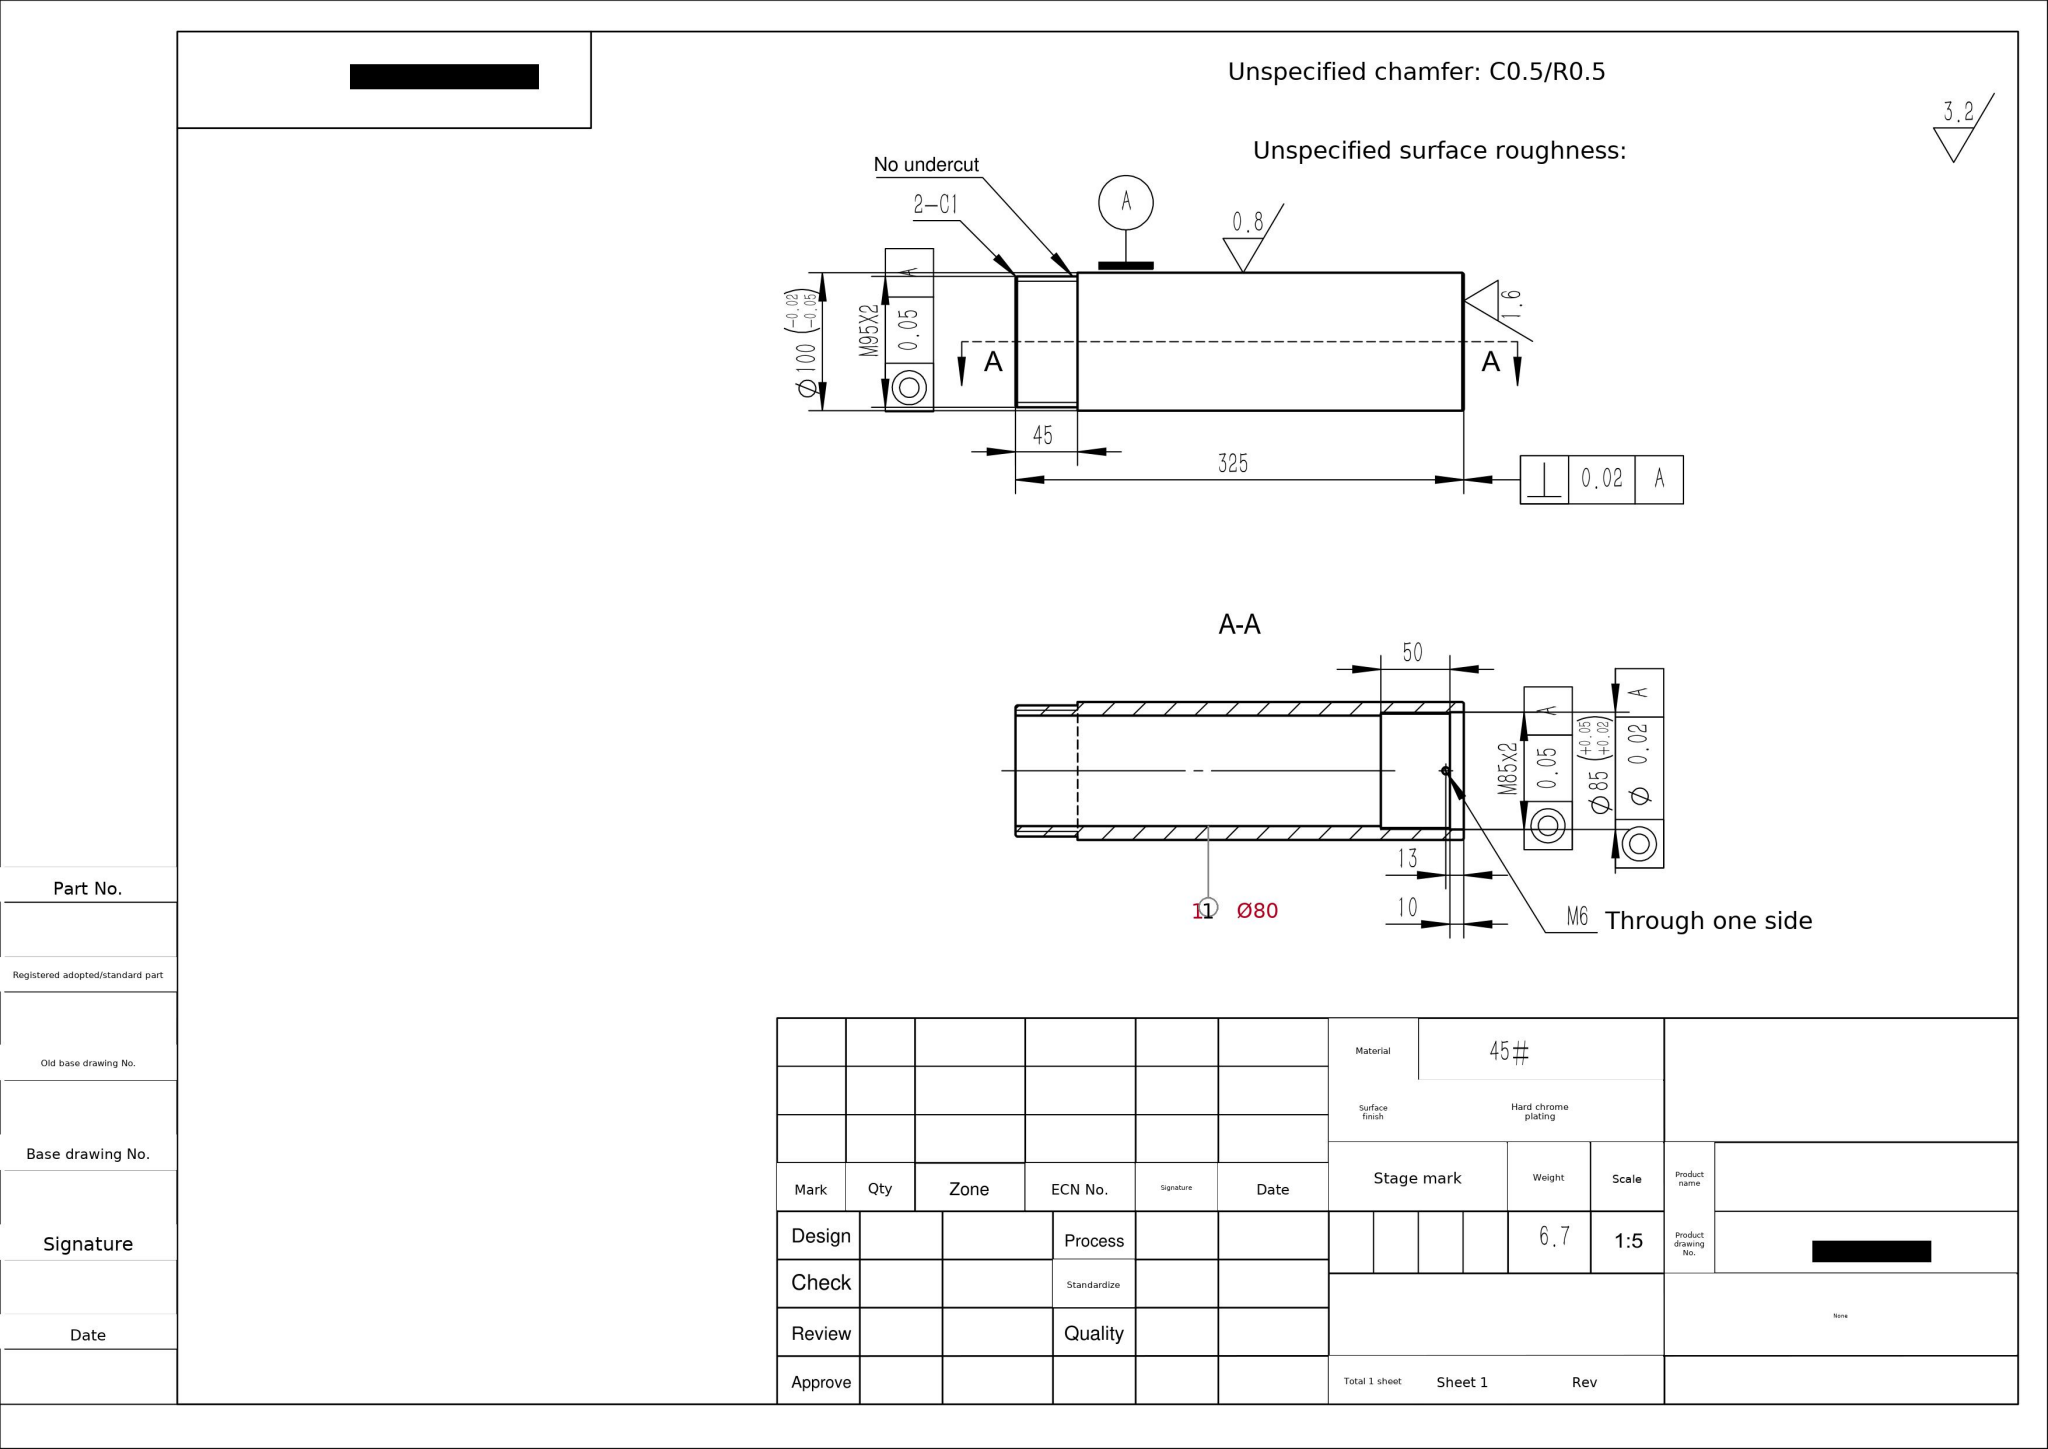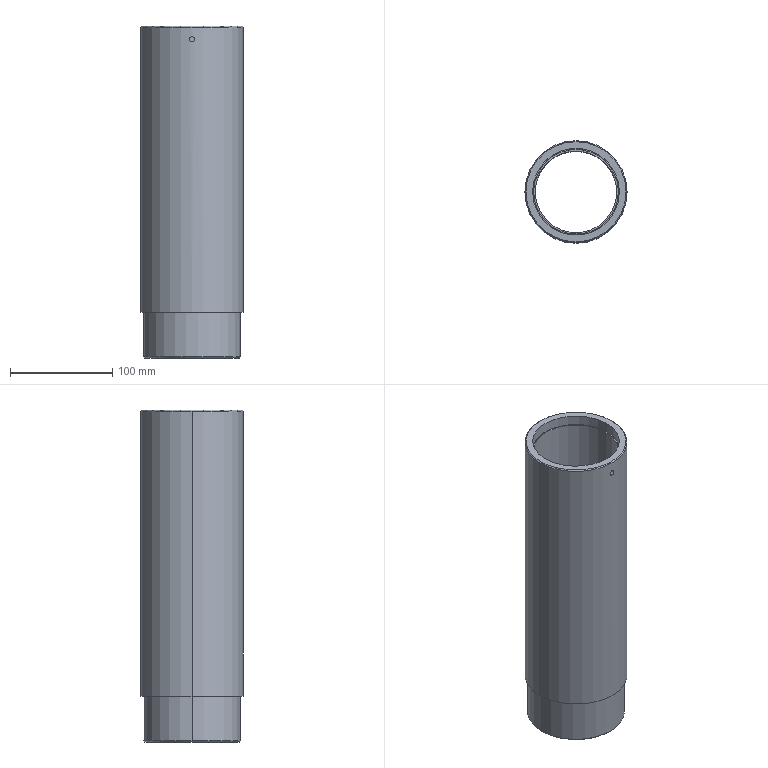Part | SolidWorks | mm | material 45# | 1 solid | 21 faces | box 100 x 100 x 325 mm | volume 858303 mm3 | cylinder 12 | plane 5 | cone 4 | commonest cylinder face diameters 5 x2 83 x2 85 x2 95 x2 100 x2 80 x2
build123d program:
from build123d import *

# Parameters (mm, degrees)
SKETCH1_R             = 50
SKETCH1_R_2           = 40
BOSS_EXTRUDE1_DEPTH   = 325
SKETCH2_R             = 61.681
SKETCH2_R_2           = 47.5
CUT_EXTRUDE1_DEPTH    = 45
CHAMFER1_SIZE         = 1
CHAMFER2_SIZE         = 1
SKETCH10_R            = 42.5
CUT_EXTRUDE9_DEPTH    = 10
SKETCH11_R            = 41.5
CUT_EXTRUDE10_DEPTH   = 50
M6_TAPPED_HOLE1_D     = 5
M6_TAPPED_HOLE1_DEPTH = 15
M6_TAPPED_HOLE1_TIP   = 1.502


with BuildPart() as part:
    # Sketch1 → Boss-Extrude1 (new body)
    with BuildSketch(Plane.XY):
        Circle(SKETCH1_R)
        Circle(SKETCH1_R_2, mode=Mode.SUBTRACT)
    extrude(amount=BOSS_EXTRUDE1_DEPTH)

    # Sketch2 → Cut-Extrude1 (cut)
    with BuildSketch(Plane(origin=(0, 0, 0), x_dir=(-1, 0, 0), z_dir=(0, 0, -1))):
        Circle(SKETCH2_R)
        Circle(SKETCH2_R_2, mode=Mode.SUBTRACT)
    extrude(amount=-CUT_EXTRUDE1_DEPTH, mode=Mode.SUBTRACT)

    # Chamfer1
    chamfer1_edges = [part.edges().sort_by_distance(p)[0] for p in [
        (47.5, 0, 0),
    ]]
    chamfer(chamfer1_edges, length=CHAMFER1_SIZE)

    # Chamfer2
    chamfer2_edges = [part.edges().sort_by_distance(p)[0] for p in [
        (-50, 0, 325),
    ]]
    chamfer(chamfer2_edges, length=CHAMFER2_SIZE)

    # Sketch10 → Cut-Extrude9 (cut)
    with BuildSketch(Plane.XY.offset(325)):
        Circle(SKETCH10_R)
    extrude(amount=-CUT_EXTRUDE9_DEPTH, mode=Mode.SUBTRACT)

    # Sketch11 → Cut-Extrude10 (cut)
    with BuildSketch(Plane.XY.offset(315)):
        Circle(SKETCH11_R)
    extrude(amount=-CUT_EXTRUDE10_DEPTH, mode=Mode.SUBTRACT)

    # M6 Tapped Hole1
    with Locations(Plane.XZ.offset(50)):
        with Locations((0, 312)):
            Hole(M6_TAPPED_HOLE1_D / 2, depth=M6_TAPPED_HOLE1_DEPTH)
            with Locations((0, 0, -(M6_TAPPED_HOLE1_DEPTH + M6_TAPPED_HOLE1_TIP / 2))):  # 118° drill point
                Cone(0, M6_TAPPED_HOLE1_D / 2, M6_TAPPED_HOLE1_TIP, mode=Mode.SUBTRACT)


solid = part.part
STEP:
#1=CARTESIAN_POINT('',(0.,-41.5,314.5));
#2=VERTEX_POINT('',#1);
#3=CARTESIAN_POINT('',(-0.,-41.5,309.5));
#4=VERTEX_POINT('',#3);
#5=CARTESIAN_POINT('',(0.,-41.5,314.5));
#6=CARTESIAN_POINT('',(-0.1631,-41.5,314.5));
#7=CARTESIAN_POINT('',(-0.3253,-41.499,314.484));
#8=CARTESIAN_POINT('',(-0.6476,-41.495,314.42));
#9=CARTESIAN_POINT('',(-0.8056,-41.492,314.372));
#10=CARTESIAN_POINT('',(-1.257,-41.482,314.185));
#11=CARTESIAN_POINT('',(-1.536,-41.472,313.999));
#12=CARTESIAN_POINT('',(-1.882,-41.457,313.654));
#13=CARTESIAN_POINT('',(-1.987,-41.452,313.525));
#14=CARTESIAN_POINT('',(-2.169,-41.443,313.254));
#15=CARTESIAN_POINT('',(-2.246,-41.439,313.11));
#16=CARTESIAN_POINT('',(-2.372,-41.432,312.808));
#17=CARTESIAN_POINT('',(-2.42,-41.429,312.649));
#18=CARTESIAN_POINT('',(-2.484,-41.426,312.329));
#19=CARTESIAN_POINT('',(-2.5,-41.425,312.167));
#20=CARTESIAN_POINT('',(-2.5,-41.425,311.837));
#21=CARTESIAN_POINT('',(-2.484,-41.426,311.674));
#22=CARTESIAN_POINT('',(-2.421,-41.429,311.355));
#23=CARTESIAN_POINT('',(-2.373,-41.432,311.196));
#24=CARTESIAN_POINT('',(-2.248,-41.439,310.893));
#25=CARTESIAN_POINT('',(-2.171,-41.443,310.749));
#26=CARTESIAN_POINT('',(-1.99,-41.452,310.478));
#27=CARTESIAN_POINT('',(-1.884,-41.457,310.349));
#28=CARTESIAN_POINT('',(-1.654,-41.467,310.118));
#29=CARTESIAN_POINT('',(-1.528,-41.472,310.015));
#30=CARTESIAN_POINT('',(-1.255,-41.481,309.832));
#31=CARTESIAN_POINT('',(-1.11,-41.485,309.754));
#32=CARTESIAN_POINT('',(-0.6586,-41.496,309.566));
#33=CARTESIAN_POINT('',(-0.3304,-41.5,309.5));
#34=CARTESIAN_POINT('',(-0.,-41.5,309.5));
#35=B_SPLINE_CURVE_WITH_KNOTS('',3,(#5,#6,#7,#8,#9,#10,#11,#12,#13,#14,#15,#16,#17,#18,#19,#20,#21,#22,#23,#24,#25,#26,#27,#28,#29,#30,#31,#32,#33,#34),.UNSPECIFIED.,.F.,.F.,(4,2,2,2,2,2,2,2,2,2,2,2,2,2,4),(0.007818,0.008306,0.008795,0.009772,0.01026,0.01075,0.01124,0.01173,0.01221,0.0127,0.01319,0.01368,0.01417,0.01466,0.01563),.UNSPECIFIED.);
#36=EDGE_CURVE('',#2,#4,#35,.T.);
#37=ORIENTED_EDGE('',*,*,#36,.F.);
#38=CARTESIAN_POINT('',(0.,-50.,314.5));
#39=VERTEX_POINT('',#38);
#40=CARTESIAN_POINT('',(0.,-50.,314.5));
#41=DIRECTION('',(0.,-1.,0.));
#42=VECTOR('',#41,1000.);
#43=LINE('',#40,#42);
#44=EDGE_CURVE('',#2,#39,#43,.T.);
#45=ORIENTED_EDGE('',*,*,#44,.T.);
#46=CARTESIAN_POINT('',(-0.,-50.,309.5));
#47=VERTEX_POINT('',#46);
#48=CARTESIAN_POINT('',(-0.,-50.,309.5));
#49=CARTESIAN_POINT('',(-0.1652,-50.,309.5));
#50=CARTESIAN_POINT('',(-0.3277,-49.999,309.516));
#51=CARTESIAN_POINT('',(-0.6472,-49.996,309.58));
#52=CARTESIAN_POINT('',(-0.806,-49.994,309.628));
#53=CARTESIAN_POINT('',(-1.109,-49.988,309.753));
#54=CARTESIAN_POINT('',(-1.252,-49.984,309.83));
#55=CARTESIAN_POINT('',(-1.524,-49.977,310.012));
#56=CARTESIAN_POINT('',(-1.653,-49.973,310.117));
#57=CARTESIAN_POINT('',(-1.883,-49.965,310.348));
#58=CARTESIAN_POINT('',(-1.987,-49.961,310.474));
#59=CARTESIAN_POINT('',(-2.17,-49.953,310.747));
#60=CARTESIAN_POINT('',(-2.247,-49.95,310.893));
#61=CARTESIAN_POINT('',(-2.372,-49.944,311.193));
#62=CARTESIAN_POINT('',(-2.42,-49.941,311.351));
#63=CARTESIAN_POINT('',(-2.484,-49.938,311.674));
#64=CARTESIAN_POINT('',(-2.5,-49.937,311.836));
#65=CARTESIAN_POINT('',(-2.5,-49.937,312.162));
#66=CARTESIAN_POINT('',(-2.484,-49.938,312.328));
#67=CARTESIAN_POINT('',(-2.42,-49.941,312.649));
#68=CARTESIAN_POINT('',(-2.373,-49.944,312.804));
#69=CARTESIAN_POINT('',(-2.247,-49.95,313.107));
#70=CARTESIAN_POINT('',(-2.169,-49.953,313.253));
#71=CARTESIAN_POINT('',(-1.988,-49.961,313.524));
#72=CARTESIAN_POINT('',(-1.885,-49.965,313.651));
#73=CARTESIAN_POINT('',(-1.651,-49.973,313.884));
#74=CARTESIAN_POINT('',(-1.525,-49.977,313.988));
#75=CARTESIAN_POINT('',(-1.254,-49.984,314.169));
#76=CARTESIAN_POINT('',(-1.108,-49.988,314.247));
#77=CARTESIAN_POINT('',(-0.8052,-49.994,314.372));
#78=CARTESIAN_POINT('',(-0.6493,-49.996,314.42));
#79=CARTESIAN_POINT('',(-0.3289,-49.999,314.484));
#80=CARTESIAN_POINT('',(-0.1632,-50.,314.5));
#81=CARTESIAN_POINT('',(0.,-50.,314.5));
#82=B_SPLINE_CURVE_WITH_KNOTS('',3,(#48,#49,#50,#51,#52,#53,#54,#55,#56,#57,#58,#59,#60,#61,#62,#63,#64,#65,#66,#67,#68,#69,#70,#71,#72,#73,#74,#75,#76,#77,#78,#79,#80,#81),.UNSPECIFIED.,.F.,.F.,(4,2,2,2,2,2,2,2,2,2,2,2,2,2,2,2,4),(0.,0.0004886,0.0009772,0.001466,0.001954,0.002443,0.002932,0.00342,0.003909,0.004397,0.004886,0.005374,0.005863,0.006352,0.00684,0.007329,0.007817),.UNSPECIFIED.);
#83=EDGE_CURVE('',#47,#39,#82,.T.);
#84=ORIENTED_EDGE('',*,*,#83,.F.);
#85=CARTESIAN_POINT('',(0.,-50.,309.5));
#86=DIRECTION('',(0.,-1.,0.));
#87=VECTOR('',#86,1000.);
#88=LINE('',#85,#87);
#89=EDGE_CURVE('',#4,#47,#88,.T.);
#90=ORIENTED_EDGE('',*,*,#89,.F.);
#91=EDGE_LOOP('',(#37,#45,#84,#90));
#92=FACE_OUTER_BOUND('',#91,.T.);
#93=CARTESIAN_POINT('',(0.,-50.,312.));
#94=DIRECTION('',(0.,-1.,0.));
#95=DIRECTION('',(0.,0.,-1.));
#96=AXIS2_PLACEMENT_3D('',#93,#94,#95);
#97=CYLINDRICAL_SURFACE('',#96,2.5);
#98=ADVANCED_FACE('',(#92),#97,.F.);
#99=CARTESIAN_POINT('',(-0.,-41.5,309.5));
#100=CARTESIAN_POINT('',(0.1652,-41.5,309.5));
#101=CARTESIAN_POINT('',(0.3277,-41.499,309.516));
#102=CARTESIAN_POINT('',(0.6473,-41.495,309.58));
#103=CARTESIAN_POINT('',(0.8061,-41.492,309.628));
#104=CARTESIAN_POINT('',(1.109,-41.485,309.753));
#105=CARTESIAN_POINT('',(1.252,-41.481,309.83));
#106=CARTESIAN_POINT('',(1.524,-41.472,310.012));
#107=CARTESIAN_POINT('',(1.653,-41.467,310.117));
#108=CARTESIAN_POINT('',(1.883,-41.457,310.348));
#109=CARTESIAN_POINT('',(1.987,-41.453,310.474));
#110=CARTESIAN_POINT('',(2.17,-41.443,310.747));
#111=CARTESIAN_POINT('',(2.247,-41.439,310.893));
#112=CARTESIAN_POINT('',(2.372,-41.432,311.193));
#113=CARTESIAN_POINT('',(2.42,-41.429,311.351));
#114=CARTESIAN_POINT('',(2.484,-41.426,311.674));
#115=CARTESIAN_POINT('',(2.5,-41.425,311.836));
#116=CARTESIAN_POINT('',(2.5,-41.425,312.162));
#117=CARTESIAN_POINT('',(2.484,-41.426,312.328));
#118=CARTESIAN_POINT('',(2.42,-41.429,312.649));
#119=CARTESIAN_POINT('',(2.373,-41.432,312.804));
#120=CARTESIAN_POINT('',(2.247,-41.439,313.107));
#121=CARTESIAN_POINT('',(2.169,-41.443,313.254));
#122=CARTESIAN_POINT('',(1.988,-41.452,313.524));
#123=CARTESIAN_POINT('',(1.885,-41.457,313.651));
#124=CARTESIAN_POINT('',(1.651,-41.467,313.884));
#125=CARTESIAN_POINT('',(1.525,-41.472,313.988));
#126=CARTESIAN_POINT('',(1.254,-41.481,314.169));
#127=CARTESIAN_POINT('',(1.108,-41.485,314.247));
#128=CARTESIAN_POINT('',(0.8052,-41.492,314.372));
#129=CARTESIAN_POINT('',(0.6493,-41.495,314.42));
#130=CARTESIAN_POINT('',(0.3289,-41.499,314.484));
#131=CARTESIAN_POINT('',(0.1632,-41.5,314.5));
#132=CARTESIAN_POINT('',(0.,-41.5,314.5));
#133=B_SPLINE_CURVE_WITH_KNOTS('',3,(#99,#100,#101,#102,#103,#104,#105,#106,#107,#108,#109,#110,#111,#112,#113,#114,#115,#116,#117,#118,#119,#120,#121,#122,#123,#124,#125,#126,#127,#128,#129,#130,#131,#132),.UNSPECIFIED.,.F.,.F.,(4,2,2,2,2,2,2,2,2,2,2,2,2,2,2,2,4),(0.,0.0004886,0.0009772,0.001466,0.001954,0.002443,0.002932,0.00342,0.003909,0.004398,0.004886,0.005375,0.005863,0.006352,0.006841,0.007329,0.007818),.UNSPECIFIED.);
#134=EDGE_CURVE('',#4,#2,#133,.T.);
#135=ORIENTED_EDGE('',*,*,#134,.T.);
#136=ORIENTED_EDGE('',*,*,#36,.T.);
#137=EDGE_LOOP('',(#135,#136));
#138=FACE_BOUND('',#137,.T.);
#139=CARTESIAN_POINT('',(-41.5,0.,265.));
#140=VERTEX_POINT('',#139);
#141=CARTESIAN_POINT('',(41.5,0.,265.));
#142=VERTEX_POINT('',#141);
#143=CARTESIAN_POINT('',(0.,0.,265.));
#144=DIRECTION('',(0.,0.,1.));
#145=DIRECTION('',(1.,0.,0.));
#146=AXIS2_PLACEMENT_3D('',#143,#144,#145);
#147=CIRCLE('',#146,41.5);
#148=EDGE_CURVE('',#140,#142,#147,.T.);
#149=ORIENTED_EDGE('',*,*,#148,.F.);
#150=CARTESIAN_POINT('',(-41.5,0.,315.));
#151=VERTEX_POINT('',#150);
#152=CARTESIAN_POINT('',(-41.5,0.,265.));
#153=DIRECTION('',(0.,0.,1.));
#154=VECTOR('',#153,1000.);
#155=LINE('',#152,#154);
#156=EDGE_CURVE('',#140,#151,#155,.T.);
#157=ORIENTED_EDGE('',*,*,#156,.T.);
#158=CARTESIAN_POINT('',(41.5,0.,315.));
#159=VERTEX_POINT('',#158);
#160=CARTESIAN_POINT('',(0.,0.,315.));
#161=DIRECTION('',(0.,0.,1.));
#162=DIRECTION('',(1.,0.,0.));
#163=AXIS2_PLACEMENT_3D('',#160,#161,#162);
#164=CIRCLE('',#163,41.5);
#165=EDGE_CURVE('',#151,#159,#164,.T.);
#166=ORIENTED_EDGE('',*,*,#165,.T.);
#167=CARTESIAN_POINT('',(41.5,0.,265.));
#168=DIRECTION('',(0.,0.,1.));
#169=VECTOR('',#168,1000.);
#170=LINE('',#167,#169);
#171=EDGE_CURVE('',#142,#159,#170,.T.);
#172=ORIENTED_EDGE('',*,*,#171,.F.);
#173=EDGE_LOOP('',(#149,#157,#166,#172));
#174=FACE_OUTER_BOUND('',#173,.T.);
#175=CARTESIAN_POINT('',(0.,0.,265.));
#176=DIRECTION('',(0.,0.,1.));
#177=DIRECTION('',(1.,0.,0.));
#178=AXIS2_PLACEMENT_3D('',#175,#176,#177);
#179=CYLINDRICAL_SURFACE('',#178,41.5);
#180=ADVANCED_FACE('',(#138,#174),#179,.F.);
#181=CARTESIAN_POINT('',(-42.5,0.,315.));
#182=VERTEX_POINT('',#181);
#183=CARTESIAN_POINT('',(42.5,0.,315.));
#184=VERTEX_POINT('',#183);
#185=CARTESIAN_POINT('',(0.,0.,315.));
#186=DIRECTION('',(0.,0.,1.));
#187=DIRECTION('',(1.,0.,0.));
#188=AXIS2_PLACEMENT_3D('',#185,#186,#187);
#189=CIRCLE('',#188,42.5);
#190=EDGE_CURVE('',#182,#184,#189,.T.);
#191=ORIENTED_EDGE('',*,*,#190,.F.);
#192=CARTESIAN_POINT('',(-42.5,0.,325.));
#193=VERTEX_POINT('',#192);
#194=CARTESIAN_POINT('',(-42.5,0.,315.));
#195=DIRECTION('',(0.,0.,1.));
#196=VECTOR('',#195,1000.);
#197=LINE('',#194,#196);
#198=EDGE_CURVE('',#182,#193,#197,.T.);
#199=ORIENTED_EDGE('',*,*,#198,.T.);
#200=CARTESIAN_POINT('',(42.5,0.,325.));
#201=VERTEX_POINT('',#200);
#202=CARTESIAN_POINT('',(0.,0.,325.));
#203=DIRECTION('',(0.,0.,1.));
#204=DIRECTION('',(1.,0.,0.));
#205=AXIS2_PLACEMENT_3D('',#202,#203,#204);
#206=CIRCLE('',#205,42.5);
#207=EDGE_CURVE('',#193,#201,#206,.T.);
#208=ORIENTED_EDGE('',*,*,#207,.T.);
#209=CARTESIAN_POINT('',(42.5,0.,315.));
#210=DIRECTION('',(0.,0.,1.));
#211=VECTOR('',#210,1000.);
#212=LINE('',#209,#211);
#213=EDGE_CURVE('',#184,#201,#212,.T.);
#214=ORIENTED_EDGE('',*,*,#213,.F.);
#215=EDGE_LOOP('',(#191,#199,#208,#214));
#216=FACE_OUTER_BOUND('',#215,.T.);
#217=CARTESIAN_POINT('',(0.,0.,315.));
#218=DIRECTION('',(0.,0.,1.));
#219=DIRECTION('',(1.,0.,0.));
#220=AXIS2_PLACEMENT_3D('',#217,#218,#219);
#221=CYLINDRICAL_SURFACE('',#220,42.5);
#222=ADVANCED_FACE('',(#216),#221,.F.);
#223=CARTESIAN_POINT('',(49.,0.,325.));
#224=VERTEX_POINT('',#223);
#225=CARTESIAN_POINT('',(-49.,0.,325.));
#226=VERTEX_POINT('',#225);
#227=CARTESIAN_POINT('',(0.,0.,325.));
#228=DIRECTION('',(0.,0.,1.));
#229=DIRECTION('',(1.,0.,0.));
#230=AXIS2_PLACEMENT_3D('',#227,#228,#229);
#231=CIRCLE('',#230,49.);
#232=EDGE_CURVE('',#224,#226,#231,.T.);
#233=ORIENTED_EDGE('',*,*,#232,.F.);
#234=CARTESIAN_POINT('',(50.,0.,324.));
#235=VERTEX_POINT('',#234);
#236=CARTESIAN_POINT('',(49.,0.,325.));
#237=DIRECTION('',(0.7071,0.,-0.7071));
#238=VECTOR('',#237,1000.);
#239=LINE('',#236,#238);
#240=EDGE_CURVE('',#224,#235,#239,.T.);
#241=ORIENTED_EDGE('',*,*,#240,.T.);
#242=CARTESIAN_POINT('',(-50.,0.,324.));
#243=VERTEX_POINT('',#242);
#244=CARTESIAN_POINT('',(0.,0.,324.));
#245=DIRECTION('',(0.,0.,-1.));
#246=DIRECTION('',(1.,0.,0.));
#247=AXIS2_PLACEMENT_3D('',#244,#245,#246);
#248=CIRCLE('',#247,50.);
#249=EDGE_CURVE('',#243,#235,#248,.T.);
#250=ORIENTED_EDGE('',*,*,#249,.F.);
#251=CARTESIAN_POINT('',(-49.,0.,325.));
#252=DIRECTION('',(-0.7071,0.,-0.7071));
#253=VECTOR('',#252,1000.);
#254=LINE('',#251,#253);
#255=EDGE_CURVE('',#226,#243,#254,.T.);
#256=ORIENTED_EDGE('',*,*,#255,.F.);
#257=EDGE_LOOP('',(#233,#241,#250,#256));
#258=FACE_OUTER_BOUND('',#257,.T.);
#259=CARTESIAN_POINT('',(0.,0.,325.));
#260=DIRECTION('',(0.,0.,-1.));
#261=DIRECTION('',(-1.,0.,0.));
#262=AXIS2_PLACEMENT_3D('',#259,#260,#261);
#263=CONICAL_SURFACE('',#262,49.,0.7854);
#264=ADVANCED_FACE('',(#258),#263,.T.);
#265=CARTESIAN_POINT('',(-46.5,0.,0.));
#266=VERTEX_POINT('',#265);
#267=CARTESIAN_POINT('',(46.5,0.,0.));
#268=VERTEX_POINT('',#267);
#269=CARTESIAN_POINT('',(0.,0.,0.));
#270=DIRECTION('',(0.,0.,-1.));
#271=DIRECTION('',(1.,0.,0.));
#272=AXIS2_PLACEMENT_3D('',#269,#270,#271);
#273=CIRCLE('',#272,46.5);
#274=EDGE_CURVE('',#266,#268,#273,.T.);
#275=ORIENTED_EDGE('',*,*,#274,.F.);
#276=CARTESIAN_POINT('',(-47.5,0.,1.));
#277=VERTEX_POINT('',#276);
#278=CARTESIAN_POINT('',(-46.5,0.,0.));
#279=DIRECTION('',(-0.7071,0.,0.7071));
#280=VECTOR('',#279,1000.);
#281=LINE('',#278,#280);
#282=EDGE_CURVE('',#266,#277,#281,.T.);
#283=ORIENTED_EDGE('',*,*,#282,.T.);
#284=CARTESIAN_POINT('',(47.5,0.,1.));
#285=VERTEX_POINT('',#284);
#286=CARTESIAN_POINT('',(0.,0.,1.));
#287=DIRECTION('',(0.,0.,1.));
#288=DIRECTION('',(1.,0.,0.));
#289=AXIS2_PLACEMENT_3D('',#286,#287,#288);
#290=CIRCLE('',#289,47.5);
#291=EDGE_CURVE('',#285,#277,#290,.T.);
#292=ORIENTED_EDGE('',*,*,#291,.F.);
#293=CARTESIAN_POINT('',(46.5,0.,0.));
#294=DIRECTION('',(0.7071,0.,0.7071));
#295=VECTOR('',#294,1000.);
#296=LINE('',#293,#295);
#297=EDGE_CURVE('',#268,#285,#296,.T.);
#298=ORIENTED_EDGE('',*,*,#297,.F.);
#299=EDGE_LOOP('',(#275,#283,#292,#298));
#300=FACE_OUTER_BOUND('',#299,.T.);
#301=CARTESIAN_POINT('',(0.,0.,0.));
#302=DIRECTION('',(0.,0.,1.));
#303=DIRECTION('',(1.,0.,0.));
#304=AXIS2_PLACEMENT_3D('',#301,#302,#303);
#305=CONICAL_SURFACE('',#304,46.5,0.7854);
#306=ADVANCED_FACE('',(#300),#305,.T.);
#307=CARTESIAN_POINT('',(-47.5,0.,45.));
#308=VERTEX_POINT('',#307);
#309=CARTESIAN_POINT('',(47.5,0.,45.));
#310=VERTEX_POINT('',#309);
#311=CARTESIAN_POINT('',(0.,0.,45.));
#312=DIRECTION('',(0.,0.,-1.));
#313=DIRECTION('',(-1.,0.,0.));
#314=AXIS2_PLACEMENT_3D('',#311,#312,#313);
#315=CIRCLE('',#314,47.5);
#316=EDGE_CURVE('',#308,#310,#315,.T.);
#317=ORIENTED_EDGE('',*,*,#316,.T.);
#318=CARTESIAN_POINT('',(47.5,0.,45.));
#319=DIRECTION('',(0.,0.,-1.));
#320=VECTOR('',#319,1000.);
#321=LINE('',#318,#320);
#322=EDGE_CURVE('',#310,#285,#321,.T.);
#323=ORIENTED_EDGE('',*,*,#322,.T.);
#324=ORIENTED_EDGE('',*,*,#291,.T.);
#325=CARTESIAN_POINT('',(-47.5,0.,45.));
#326=DIRECTION('',(0.,0.,-1.));
#327=VECTOR('',#326,1000.);
#328=LINE('',#325,#327);
#329=EDGE_CURVE('',#308,#277,#328,.T.);
#330=ORIENTED_EDGE('',*,*,#329,.F.);
#331=EDGE_LOOP('',(#317,#323,#324,#330));
#332=FACE_OUTER_BOUND('',#331,.T.);
#333=CARTESIAN_POINT('',(0.,0.,45.));
#334=DIRECTION('',(0.,0.,-1.));
#335=DIRECTION('',(-1.,0.,0.));
#336=AXIS2_PLACEMENT_3D('',#333,#334,#335);
#337=CYLINDRICAL_SURFACE('',#336,47.5);
#338=ADVANCED_FACE('',(#332),#337,.T.);
#339=ORIENTED_EDGE('',*,*,#249,.T.);
#340=CARTESIAN_POINT('',(50.,0.,45.));
#341=VERTEX_POINT('',#340);
#342=CARTESIAN_POINT('',(50.,0.,325.));
#343=DIRECTION('',(0.,0.,-1.));
#344=VECTOR('',#343,1000.);
#345=LINE('',#342,#344);
#346=EDGE_CURVE('',#235,#341,#345,.T.);
#347=ORIENTED_EDGE('',*,*,#346,.T.);
#348=CARTESIAN_POINT('',(-50.,0.,45.));
#349=VERTEX_POINT('',#348);
#350=CARTESIAN_POINT('',(0.,0.,45.));
#351=DIRECTION('',(0.,0.,-1.));
#352=DIRECTION('',(-1.,0.,0.));
#353=AXIS2_PLACEMENT_3D('',#350,#351,#352);
#354=CIRCLE('',#353,50.);
#355=EDGE_CURVE('',#349,#341,#354,.T.);
#356=ORIENTED_EDGE('',*,*,#355,.F.);
#357=CARTESIAN_POINT('',(-50.,0.,325.));
#358=DIRECTION('',(0.,0.,-1.));
#359=VECTOR('',#358,1000.);
#360=LINE('',#357,#359);
#361=EDGE_CURVE('',#243,#349,#360,.T.);
#362=ORIENTED_EDGE('',*,*,#361,.F.);
#363=EDGE_LOOP('',(#339,#347,#356,#362));
#364=FACE_OUTER_BOUND('',#363,.T.);
#365=CARTESIAN_POINT('',(0.,0.,325.));
#366=DIRECTION('',(0.,0.,-1.));
#367=DIRECTION('',(-1.,0.,0.));
#368=AXIS2_PLACEMENT_3D('',#365,#366,#367);
#369=CYLINDRICAL_SURFACE('',#368,50.);
#370=ADVANCED_FACE('',(#364),#369,.T.);
#371=CARTESIAN_POINT('',(-40.,0.,265.));
#372=VERTEX_POINT('',#371);
#373=CARTESIAN_POINT('',(40.,0.,265.));
#374=VERTEX_POINT('',#373);
#375=CARTESIAN_POINT('',(0.,0.,265.));
#376=DIRECTION('',(0.,0.,1.));
#377=DIRECTION('',(1.,0.,0.));
#378=AXIS2_PLACEMENT_3D('',#375,#376,#377);
#379=CIRCLE('',#378,40.);
#380=EDGE_CURVE('',#372,#374,#379,.T.);
#381=ORIENTED_EDGE('',*,*,#380,.T.);
#382=CARTESIAN_POINT('',(40.,0.,0.));
#383=VERTEX_POINT('',#382);
#384=CARTESIAN_POINT('',(40.,0.,325.));
#385=DIRECTION('',(0.,0.,-1.));
#386=VECTOR('',#385,1000.);
#387=LINE('',#384,#386);
#388=EDGE_CURVE('',#374,#383,#387,.T.);
#389=ORIENTED_EDGE('',*,*,#388,.T.);
#390=CARTESIAN_POINT('',(-40.,0.,0.));
#391=VERTEX_POINT('',#390);
#392=CARTESIAN_POINT('',(0.,0.,0.));
#393=DIRECTION('',(0.,0.,1.));
#394=DIRECTION('',(1.,0.,0.));
#395=AXIS2_PLACEMENT_3D('',#392,#393,#394);
#396=CIRCLE('',#395,40.);
#397=EDGE_CURVE('',#391,#383,#396,.T.);
#398=ORIENTED_EDGE('',*,*,#397,.F.);
#399=CARTESIAN_POINT('',(-40.,0.,325.));
#400=DIRECTION('',(0.,0.,-1.));
#401=VECTOR('',#400,1000.);
#402=LINE('',#399,#401);
#403=EDGE_CURVE('',#372,#391,#402,.T.);
#404=ORIENTED_EDGE('',*,*,#403,.F.);
#405=EDGE_LOOP('',(#381,#389,#398,#404));
#406=FACE_OUTER_BOUND('',#405,.T.);
#407=CARTESIAN_POINT('',(0.,0.,325.));
#408=DIRECTION('',(0.,0.,-1.));
#409=DIRECTION('',(-1.,0.,0.));
#410=AXIS2_PLACEMENT_3D('',#407,#408,#409);
#411=CYLINDRICAL_SURFACE('',#410,40.);
#412=ADVANCED_FACE('',(#406),#411,.F.);
#413=ORIENTED_EDGE('',*,*,#388,.F.);
#414=CARTESIAN_POINT('',(0.,0.,265.));
#415=DIRECTION('',(0.,0.,1.));
#416=DIRECTION('',(1.,0.,0.));
#417=AXIS2_PLACEMENT_3D('',#414,#415,#416);
#418=CIRCLE('',#417,40.);
#419=EDGE_CURVE('',#374,#372,#418,.T.);
#420=ORIENTED_EDGE('',*,*,#419,.T.);
#421=ORIENTED_EDGE('',*,*,#403,.T.);
#422=CARTESIAN_POINT('',(0.,0.,0.));
#423=DIRECTION('',(0.,0.,1.));
#424=DIRECTION('',(1.,0.,0.));
#425=AXIS2_PLACEMENT_3D('',#422,#423,#424);
#426=CIRCLE('',#425,40.);
#427=EDGE_CURVE('',#383,#391,#426,.T.);
#428=ORIENTED_EDGE('',*,*,#427,.F.);
#429=EDGE_LOOP('',(#413,#420,#421,#428));
#430=FACE_OUTER_BOUND('',#429,.T.);
#431=CARTESIAN_POINT('',(0.,0.,325.));
#432=DIRECTION('',(0.,0.,-1.));
#433=DIRECTION('',(-1.,0.,0.));
#434=AXIS2_PLACEMENT_3D('',#431,#432,#433);
#435=CYLINDRICAL_SURFACE('',#434,40.);
#436=ADVANCED_FACE('',(#430),#435,.F.);
#437=CARTESIAN_POINT('',(0.,0.,0.));
#438=DIRECTION('',(0.,0.,-1.));
#439=DIRECTION('',(1.,0.,0.));
#440=AXIS2_PLACEMENT_3D('',#437,#438,#439);
#441=CIRCLE('',#440,46.5);
#442=EDGE_CURVE('',#268,#266,#441,.T.);
#443=ORIENTED_EDGE('',*,*,#442,.T.);
#444=ORIENTED_EDGE('',*,*,#274,.T.);
#445=EDGE_LOOP('',(#443,#444));
#446=FACE_OUTER_BOUND('',#445,.T.);
#447=ORIENTED_EDGE('',*,*,#397,.T.);
#448=ORIENTED_EDGE('',*,*,#427,.T.);
#449=EDGE_LOOP('',(#447,#448));
#450=FACE_BOUND('',#449,.T.);
#451=CARTESIAN_POINT('',(0.,0.,0.));
#452=DIRECTION('',(0.,0.,1.));
#453=DIRECTION('',(1.,0.,0.));
#454=AXIS2_PLACEMENT_3D('',#451,#452,#453);
#455=PLANE('',#454);
#456=ADVANCED_FACE('',(#446,#450),#455,.F.);
#457=ORIENTED_EDGE('',*,*,#346,.F.);
#458=CARTESIAN_POINT('',(0.,0.,324.));
#459=DIRECTION('',(0.,0.,-1.));
#460=DIRECTION('',(1.,0.,0.));
#461=AXIS2_PLACEMENT_3D('',#458,#459,#460);
#462=CIRCLE('',#461,50.);
#463=EDGE_CURVE('',#235,#243,#462,.T.);
#464=ORIENTED_EDGE('',*,*,#463,.T.);
#465=ORIENTED_EDGE('',*,*,#361,.T.);
#466=CARTESIAN_POINT('',(0.,0.,45.));
#467=DIRECTION('',(0.,0.,-1.));
#468=DIRECTION('',(-1.,0.,0.));
#469=AXIS2_PLACEMENT_3D('',#466,#467,#468);
#470=CIRCLE('',#469,50.);
#471=EDGE_CURVE('',#341,#349,#470,.T.);
#472=ORIENTED_EDGE('',*,*,#471,.F.);
#473=EDGE_LOOP('',(#457,#464,#465,#472));
#474=FACE_OUTER_BOUND('',#473,.T.);
#475=ORIENTED_EDGE('',*,*,#83,.T.);
#476=CARTESIAN_POINT('',(0.,-50.,314.5));
#477=CARTESIAN_POINT('',(0.1631,-50.,314.5));
#478=CARTESIAN_POINT('',(0.3253,-49.999,314.484));
#479=CARTESIAN_POINT('',(0.6476,-49.996,314.42));
#480=CARTESIAN_POINT('',(0.8056,-49.994,314.372));
#481=CARTESIAN_POINT('',(1.257,-49.985,314.185));
#482=CARTESIAN_POINT('',(1.536,-49.977,313.999));
#483=CARTESIAN_POINT('',(1.882,-49.965,313.654));
#484=CARTESIAN_POINT('',(1.987,-49.961,313.525));
#485=CARTESIAN_POINT('',(2.169,-49.953,313.254));
#486=CARTESIAN_POINT('',(2.246,-49.95,313.11));
#487=CARTESIAN_POINT('',(2.372,-49.944,312.808));
#488=CARTESIAN_POINT('',(2.42,-49.941,312.649));
#489=CARTESIAN_POINT('',(2.484,-49.938,312.329));
#490=CARTESIAN_POINT('',(2.5,-49.937,312.167));
#491=CARTESIAN_POINT('',(2.5,-49.937,311.837));
#492=CARTESIAN_POINT('',(2.484,-49.938,311.674));
#493=CARTESIAN_POINT('',(2.421,-49.941,311.355));
#494=CARTESIAN_POINT('',(2.373,-49.944,311.196));
#495=CARTESIAN_POINT('',(2.248,-49.949,310.893));
#496=CARTESIAN_POINT('',(2.171,-49.953,310.749));
#497=CARTESIAN_POINT('',(1.99,-49.96,310.478));
#498=CARTESIAN_POINT('',(1.884,-49.965,310.349));
#499=CARTESIAN_POINT('',(1.654,-49.973,310.118));
#500=CARTESIAN_POINT('',(1.528,-49.977,310.015));
#501=CARTESIAN_POINT('',(1.255,-49.984,309.832));
#502=CARTESIAN_POINT('',(1.11,-49.988,309.754));
#503=CARTESIAN_POINT('',(0.6585,-49.997,309.566));
#504=CARTESIAN_POINT('',(0.3303,-50.,309.5));
#505=CARTESIAN_POINT('',(-0.,-50.,309.5));
#506=B_SPLINE_CURVE_WITH_KNOTS('',3,(#476,#477,#478,#479,#480,#481,#482,#483,#484,#485,#486,#487,#488,#489,#490,#491,#492,#493,#494,#495,#496,#497,#498,#499,#500,#501,#502,#503,#504,#505),.UNSPECIFIED.,.F.,.F.,(4,2,2,2,2,2,2,2,2,2,2,2,2,2,4),(0.007817,0.008306,0.008794,0.009771,0.01026,0.01075,0.01124,0.01173,0.01221,0.0127,0.01319,0.01368,0.01417,0.01466,0.01563),.UNSPECIFIED.);
#507=EDGE_CURVE('',#39,#47,#506,.T.);
#508=ORIENTED_EDGE('',*,*,#507,.T.);
#509=EDGE_LOOP('',(#475,#508));
#510=FACE_BOUND('',#509,.T.);
#511=CARTESIAN_POINT('',(0.,0.,325.));
#512=DIRECTION('',(0.,0.,-1.));
#513=DIRECTION('',(-1.,0.,0.));
#514=AXIS2_PLACEMENT_3D('',#511,#512,#513);
#515=CYLINDRICAL_SURFACE('',#514,50.);
#516=ADVANCED_FACE('',(#474,#510),#515,.T.);
#517=CARTESIAN_POINT('',(0.,0.,325.));
#518=DIRECTION('',(0.,0.,1.));
#519=DIRECTION('',(1.,0.,0.));
#520=AXIS2_PLACEMENT_3D('',#517,#518,#519);
#521=CIRCLE('',#520,42.5);
#522=EDGE_CURVE('',#201,#193,#521,.T.);
#523=ORIENTED_EDGE('',*,*,#522,.F.);
#524=ORIENTED_EDGE('',*,*,#207,.F.);
#525=EDGE_LOOP('',(#523,#524));
#526=FACE_BOUND('',#525,.T.);
#527=CARTESIAN_POINT('',(0.,0.,325.));
#528=DIRECTION('',(0.,0.,1.));
#529=DIRECTION('',(1.,0.,0.));
#530=AXIS2_PLACEMENT_3D('',#527,#528,#529);
#531=CIRCLE('',#530,49.);
#532=EDGE_CURVE('',#226,#224,#531,.T.);
#533=ORIENTED_EDGE('',*,*,#532,.T.);
#534=ORIENTED_EDGE('',*,*,#232,.T.);
#535=EDGE_LOOP('',(#533,#534));
#536=FACE_OUTER_BOUND('',#535,.T.);
#537=CARTESIAN_POINT('',(0.,0.,325.));
#538=DIRECTION('',(0.,0.,1.));
#539=DIRECTION('',(1.,0.,0.));
#540=AXIS2_PLACEMENT_3D('',#537,#538,#539);
#541=PLANE('',#540);
#542=ADVANCED_FACE('',(#526,#536),#541,.T.);
#543=ORIENTED_EDGE('',*,*,#316,.F.);
#544=CARTESIAN_POINT('',(0.,0.,45.));
#545=DIRECTION('',(0.,0.,-1.));
#546=DIRECTION('',(-1.,0.,0.));
#547=AXIS2_PLACEMENT_3D('',#544,#545,#546);
#548=CIRCLE('',#547,47.5);
#549=EDGE_CURVE('',#310,#308,#548,.T.);
#550=ORIENTED_EDGE('',*,*,#549,.F.);
#551=EDGE_LOOP('',(#543,#550));
#552=FACE_BOUND('',#551,.T.);
#553=ORIENTED_EDGE('',*,*,#355,.T.);
#554=ORIENTED_EDGE('',*,*,#471,.T.);
#555=EDGE_LOOP('',(#553,#554));
#556=FACE_OUTER_BOUND('',#555,.T.);
#557=CARTESIAN_POINT('',(0.,0.,45.));
#558=DIRECTION('',(0.,0.,-1.));
#559=DIRECTION('',(-1.,0.,0.));
#560=AXIS2_PLACEMENT_3D('',#557,#558,#559);
#561=PLANE('',#560);
#562=ADVANCED_FACE('',(#552,#556),#561,.T.);
#563=ORIENTED_EDGE('',*,*,#322,.F.);
#564=ORIENTED_EDGE('',*,*,#549,.T.);
#565=ORIENTED_EDGE('',*,*,#329,.T.);
#566=CARTESIAN_POINT('',(0.,0.,1.));
#567=DIRECTION('',(0.,0.,1.));
#568=DIRECTION('',(1.,0.,0.));
#569=AXIS2_PLACEMENT_3D('',#566,#567,#568);
#570=CIRCLE('',#569,47.5);
#571=EDGE_CURVE('',#277,#285,#570,.T.);
#572=ORIENTED_EDGE('',*,*,#571,.T.);
#573=EDGE_LOOP('',(#563,#564,#565,#572));
#574=FACE_OUTER_BOUND('',#573,.T.);
#575=CARTESIAN_POINT('',(0.,0.,45.));
#576=DIRECTION('',(0.,0.,-1.));
#577=DIRECTION('',(-1.,0.,0.));
#578=AXIS2_PLACEMENT_3D('',#575,#576,#577);
#579=CYLINDRICAL_SURFACE('',#578,47.5);
#580=ADVANCED_FACE('',(#574),#579,.T.);
#581=ORIENTED_EDGE('',*,*,#282,.F.);
#582=ORIENTED_EDGE('',*,*,#442,.F.);
#583=ORIENTED_EDGE('',*,*,#297,.T.);
#584=ORIENTED_EDGE('',*,*,#571,.F.);
#585=EDGE_LOOP('',(#581,#582,#583,#584));
#586=FACE_OUTER_BOUND('',#585,.T.);
#587=CARTESIAN_POINT('',(0.,0.,0.));
#588=DIRECTION('',(0.,0.,1.));
#589=DIRECTION('',(1.,0.,0.));
#590=AXIS2_PLACEMENT_3D('',#587,#588,#589);
#591=CONICAL_SURFACE('',#590,46.5,0.7854);
#592=ADVANCED_FACE('',(#586),#591,.T.);
#593=ORIENTED_EDGE('',*,*,#240,.F.);
#594=ORIENTED_EDGE('',*,*,#532,.F.);
#595=ORIENTED_EDGE('',*,*,#255,.T.);
#596=ORIENTED_EDGE('',*,*,#463,.F.);
#597=EDGE_LOOP('',(#593,#594,#595,#596));
#598=FACE_OUTER_BOUND('',#597,.T.);
#599=CARTESIAN_POINT('',(0.,0.,325.));
#600=DIRECTION('',(0.,0.,-1.));
#601=DIRECTION('',(-1.,0.,0.));
#602=AXIS2_PLACEMENT_3D('',#599,#600,#601);
#603=CONICAL_SURFACE('',#602,49.,0.7854);
#604=ADVANCED_FACE('',(#598),#603,.T.);
#605=ORIENTED_EDGE('',*,*,#198,.F.);
#606=CARTESIAN_POINT('',(0.,0.,315.));
#607=DIRECTION('',(0.,0.,1.));
#608=DIRECTION('',(1.,0.,0.));
#609=AXIS2_PLACEMENT_3D('',#606,#607,#608);
#610=CIRCLE('',#609,42.5);
#611=EDGE_CURVE('',#184,#182,#610,.T.);
#612=ORIENTED_EDGE('',*,*,#611,.F.);
#613=ORIENTED_EDGE('',*,*,#213,.T.);
#614=ORIENTED_EDGE('',*,*,#522,.T.);
#615=EDGE_LOOP('',(#605,#612,#613,#614));
#616=FACE_OUTER_BOUND('',#615,.T.);
#617=CARTESIAN_POINT('',(0.,0.,315.));
#618=DIRECTION('',(0.,0.,1.));
#619=DIRECTION('',(1.,0.,0.));
#620=AXIS2_PLACEMENT_3D('',#617,#618,#619);
#621=CYLINDRICAL_SURFACE('',#620,42.5);
#622=ADVANCED_FACE('',(#616),#621,.F.);
#623=CARTESIAN_POINT('',(0.,0.,315.));
#624=DIRECTION('',(0.,0.,1.));
#625=DIRECTION('',(1.,0.,0.));
#626=AXIS2_PLACEMENT_3D('',#623,#624,#625);
#627=CIRCLE('',#626,41.5);
#628=EDGE_CURVE('',#159,#151,#627,.T.);
#629=ORIENTED_EDGE('',*,*,#628,.F.);
#630=ORIENTED_EDGE('',*,*,#165,.F.);
#631=EDGE_LOOP('',(#629,#630));
#632=FACE_BOUND('',#631,.T.);
#633=ORIENTED_EDGE('',*,*,#611,.T.);
#634=ORIENTED_EDGE('',*,*,#190,.T.);
#635=EDGE_LOOP('',(#633,#634));
#636=FACE_OUTER_BOUND('',#635,.T.);
#637=CARTESIAN_POINT('',(0.,0.,315.));
#638=DIRECTION('',(0.,0.,1.));
#639=DIRECTION('',(1.,0.,0.));
#640=AXIS2_PLACEMENT_3D('',#637,#638,#639);
#641=PLANE('',#640);
#642=ADVANCED_FACE('',(#632,#636),#641,.T.);
#643=ORIENTED_EDGE('',*,*,#156,.F.);
#644=CARTESIAN_POINT('',(0.,0.,265.));
#645=DIRECTION('',(0.,0.,1.));
#646=DIRECTION('',(1.,0.,0.));
#647=AXIS2_PLACEMENT_3D('',#644,#645,#646);
#648=CIRCLE('',#647,41.5);
#649=EDGE_CURVE('',#142,#140,#648,.T.);
#650=ORIENTED_EDGE('',*,*,#649,.F.);
#651=ORIENTED_EDGE('',*,*,#171,.T.);
#652=ORIENTED_EDGE('',*,*,#628,.T.);
#653=EDGE_LOOP('',(#643,#650,#651,#652));
#654=FACE_OUTER_BOUND('',#653,.T.);
#655=CARTESIAN_POINT('',(0.,0.,265.));
#656=DIRECTION('',(0.,0.,1.));
#657=DIRECTION('',(1.,0.,0.));
#658=AXIS2_PLACEMENT_3D('',#655,#656,#657);
#659=CYLINDRICAL_SURFACE('',#658,41.5);
#660=ADVANCED_FACE('',(#654),#659,.F.);
#661=ORIENTED_EDGE('',*,*,#380,.F.);
#662=ORIENTED_EDGE('',*,*,#419,.F.);
#663=EDGE_LOOP('',(#661,#662));
#664=FACE_BOUND('',#663,.T.);
#665=ORIENTED_EDGE('',*,*,#649,.T.);
#666=ORIENTED_EDGE('',*,*,#148,.T.);
#667=EDGE_LOOP('',(#665,#666));
#668=FACE_OUTER_BOUND('',#667,.T.);
#669=CARTESIAN_POINT('',(0.,0.,265.));
#670=DIRECTION('',(0.,0.,1.));
#671=DIRECTION('',(1.,0.,0.));
#672=AXIS2_PLACEMENT_3D('',#669,#670,#671);
#673=PLANE('',#672);
#674=ADVANCED_FACE('',(#664,#668),#673,.T.);
#675=ORIENTED_EDGE('',*,*,#44,.F.);
#676=ORIENTED_EDGE('',*,*,#134,.F.);
#677=ORIENTED_EDGE('',*,*,#89,.T.);
#678=ORIENTED_EDGE('',*,*,#507,.F.);
#679=EDGE_LOOP('',(#675,#676,#677,#678));
#680=FACE_OUTER_BOUND('',#679,.T.);
#681=CARTESIAN_POINT('',(0.,-50.,312.));
#682=DIRECTION('',(0.,-1.,0.));
#683=DIRECTION('',(0.,0.,-1.));
#684=AXIS2_PLACEMENT_3D('',#681,#682,#683);
#685=CYLINDRICAL_SURFACE('',#684,2.5);
#686=ADVANCED_FACE('',(#680),#685,.F.);
#687=CLOSED_SHELL('',(#98,#180,#222,#264,#306,#338,#370,#412,#436,#456,#516,#542,#562,#580,#592,#604,#622,#642,#660,#674,#686));
#688=MANIFOLD_SOLID_BREP('',#687);
#689=CARTESIAN_POINT('',(0.,0.,0.));
#690=DIRECTION('',(0.,0.,1.));
#691=DIRECTION('',(1.,0.,0.));
#692=AXIS2_PLACEMENT_3D('',#689,#690,#691);
#693=(LENGTH_UNIT()NAMED_UNIT(*)SI_UNIT(.MILLI.,.METRE.));
#694=UNCERTAINTY_MEASURE_WITH_UNIT(LENGTH_MEASURE(0.00001),#693,'','');
#695=(NAMED_UNIT(*)PLANE_ANGLE_UNIT()SI_UNIT($,.RADIAN.));
#696=(NAMED_UNIT(*)SI_UNIT($,.STERADIAN.)SOLID_ANGLE_UNIT());
#697=(GEOMETRIC_REPRESENTATION_CONTEXT(3)GLOBAL_UNCERTAINTY_ASSIGNED_CONTEXT((#694))GLOBAL_UNIT_ASSIGNED_CONTEXT((#693,#695,#696))REPRESENTATION_CONTEXT('',''));
#698=ADVANCED_BREP_SHAPE_REPRESENTATION('',(#688,#692),#697);